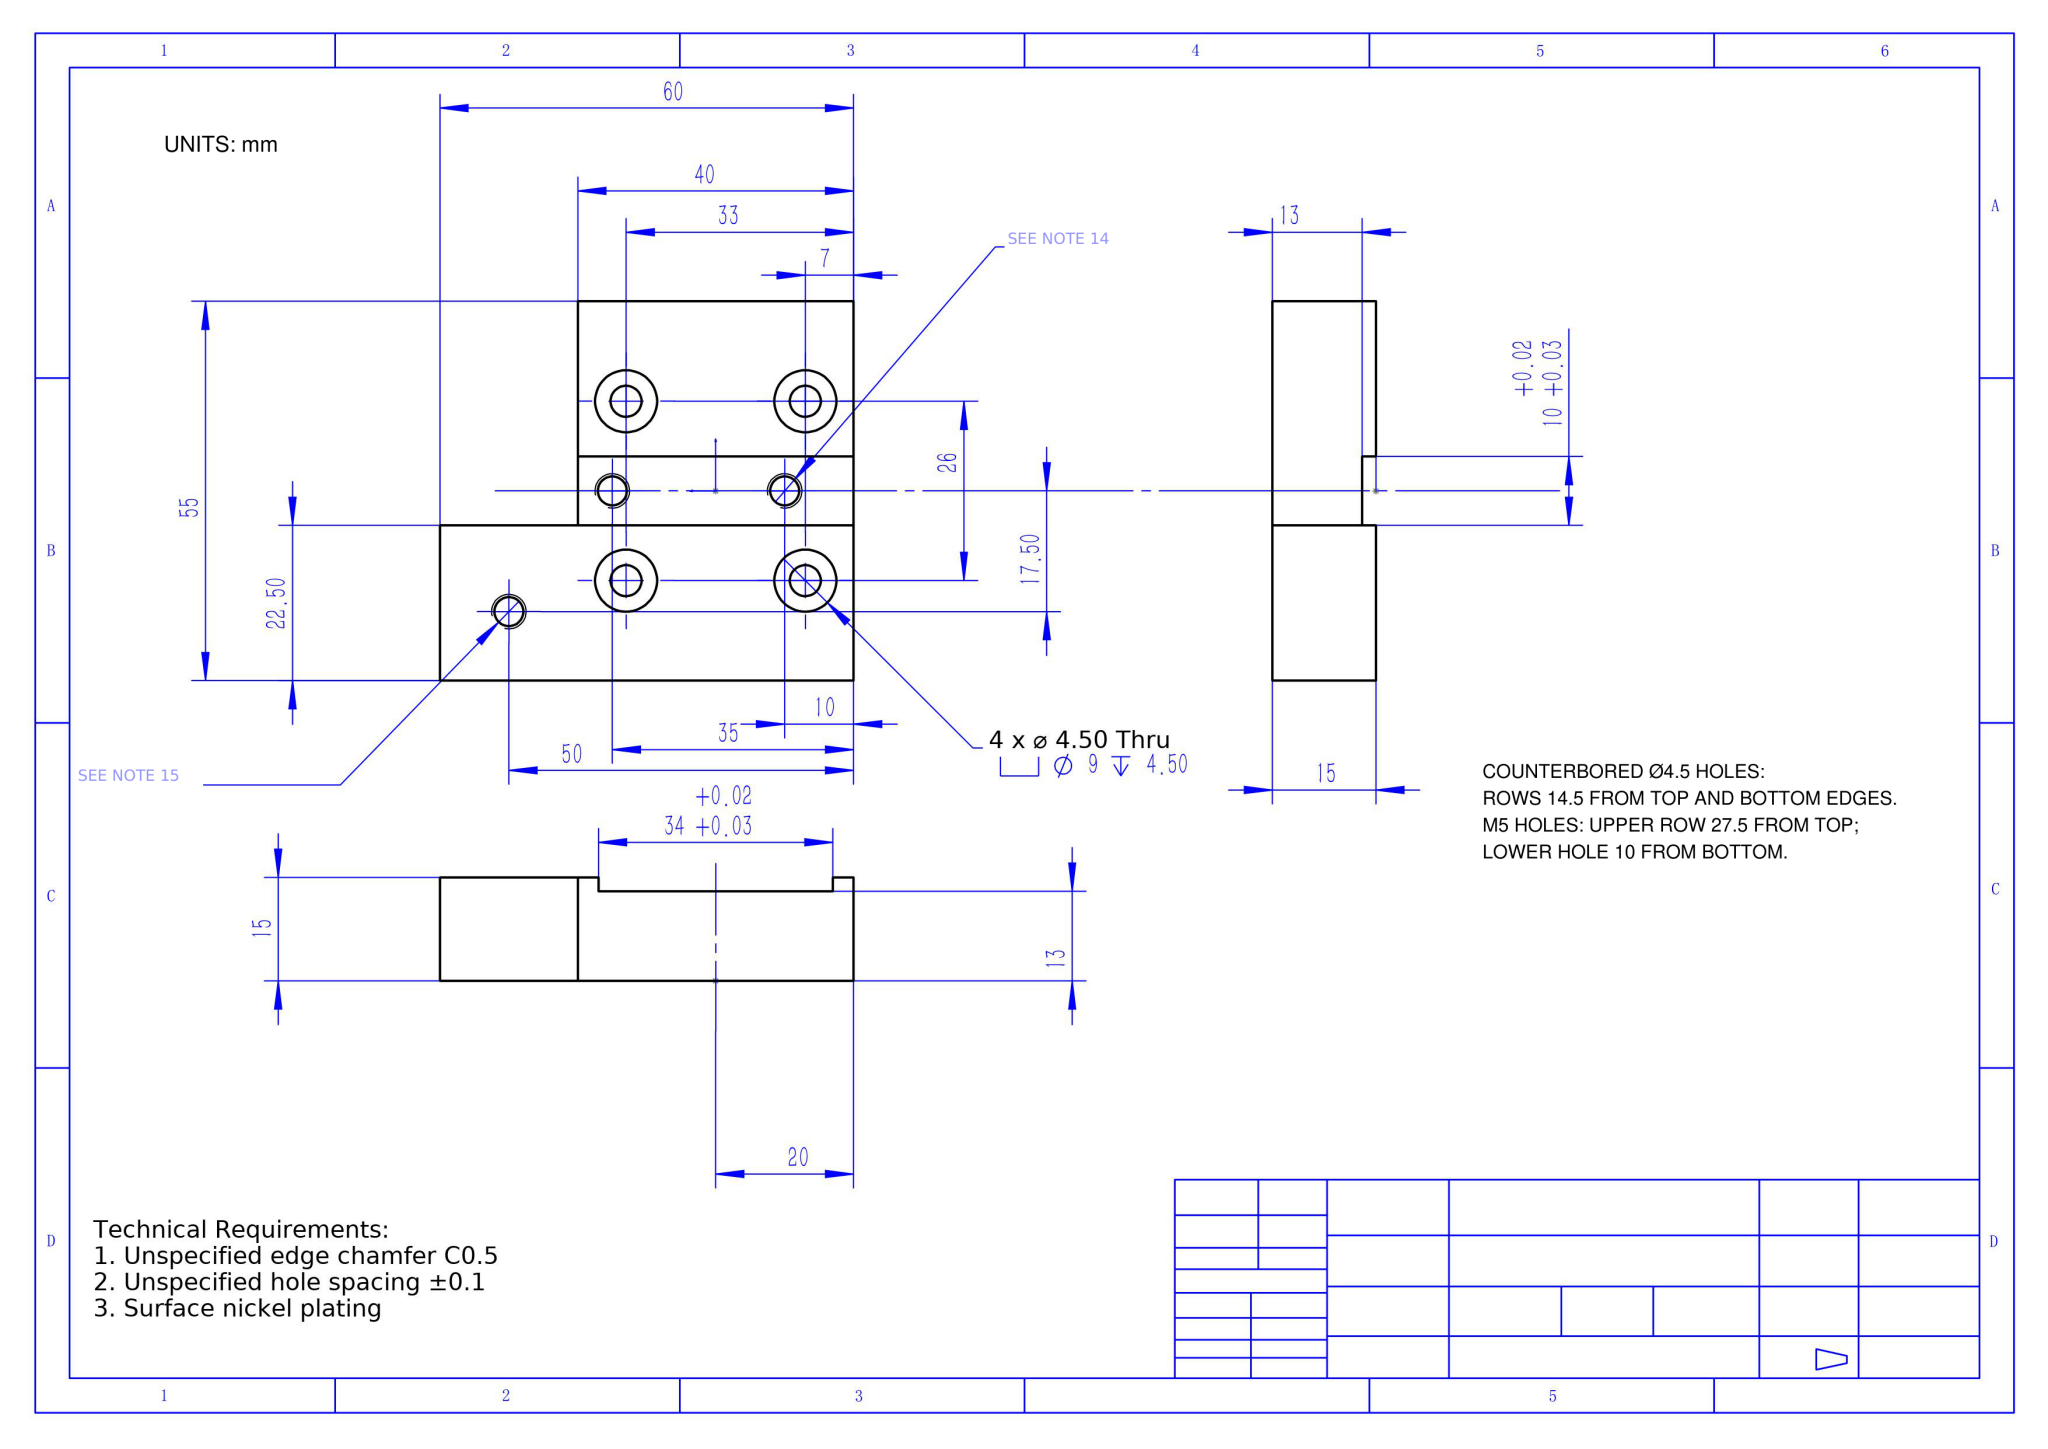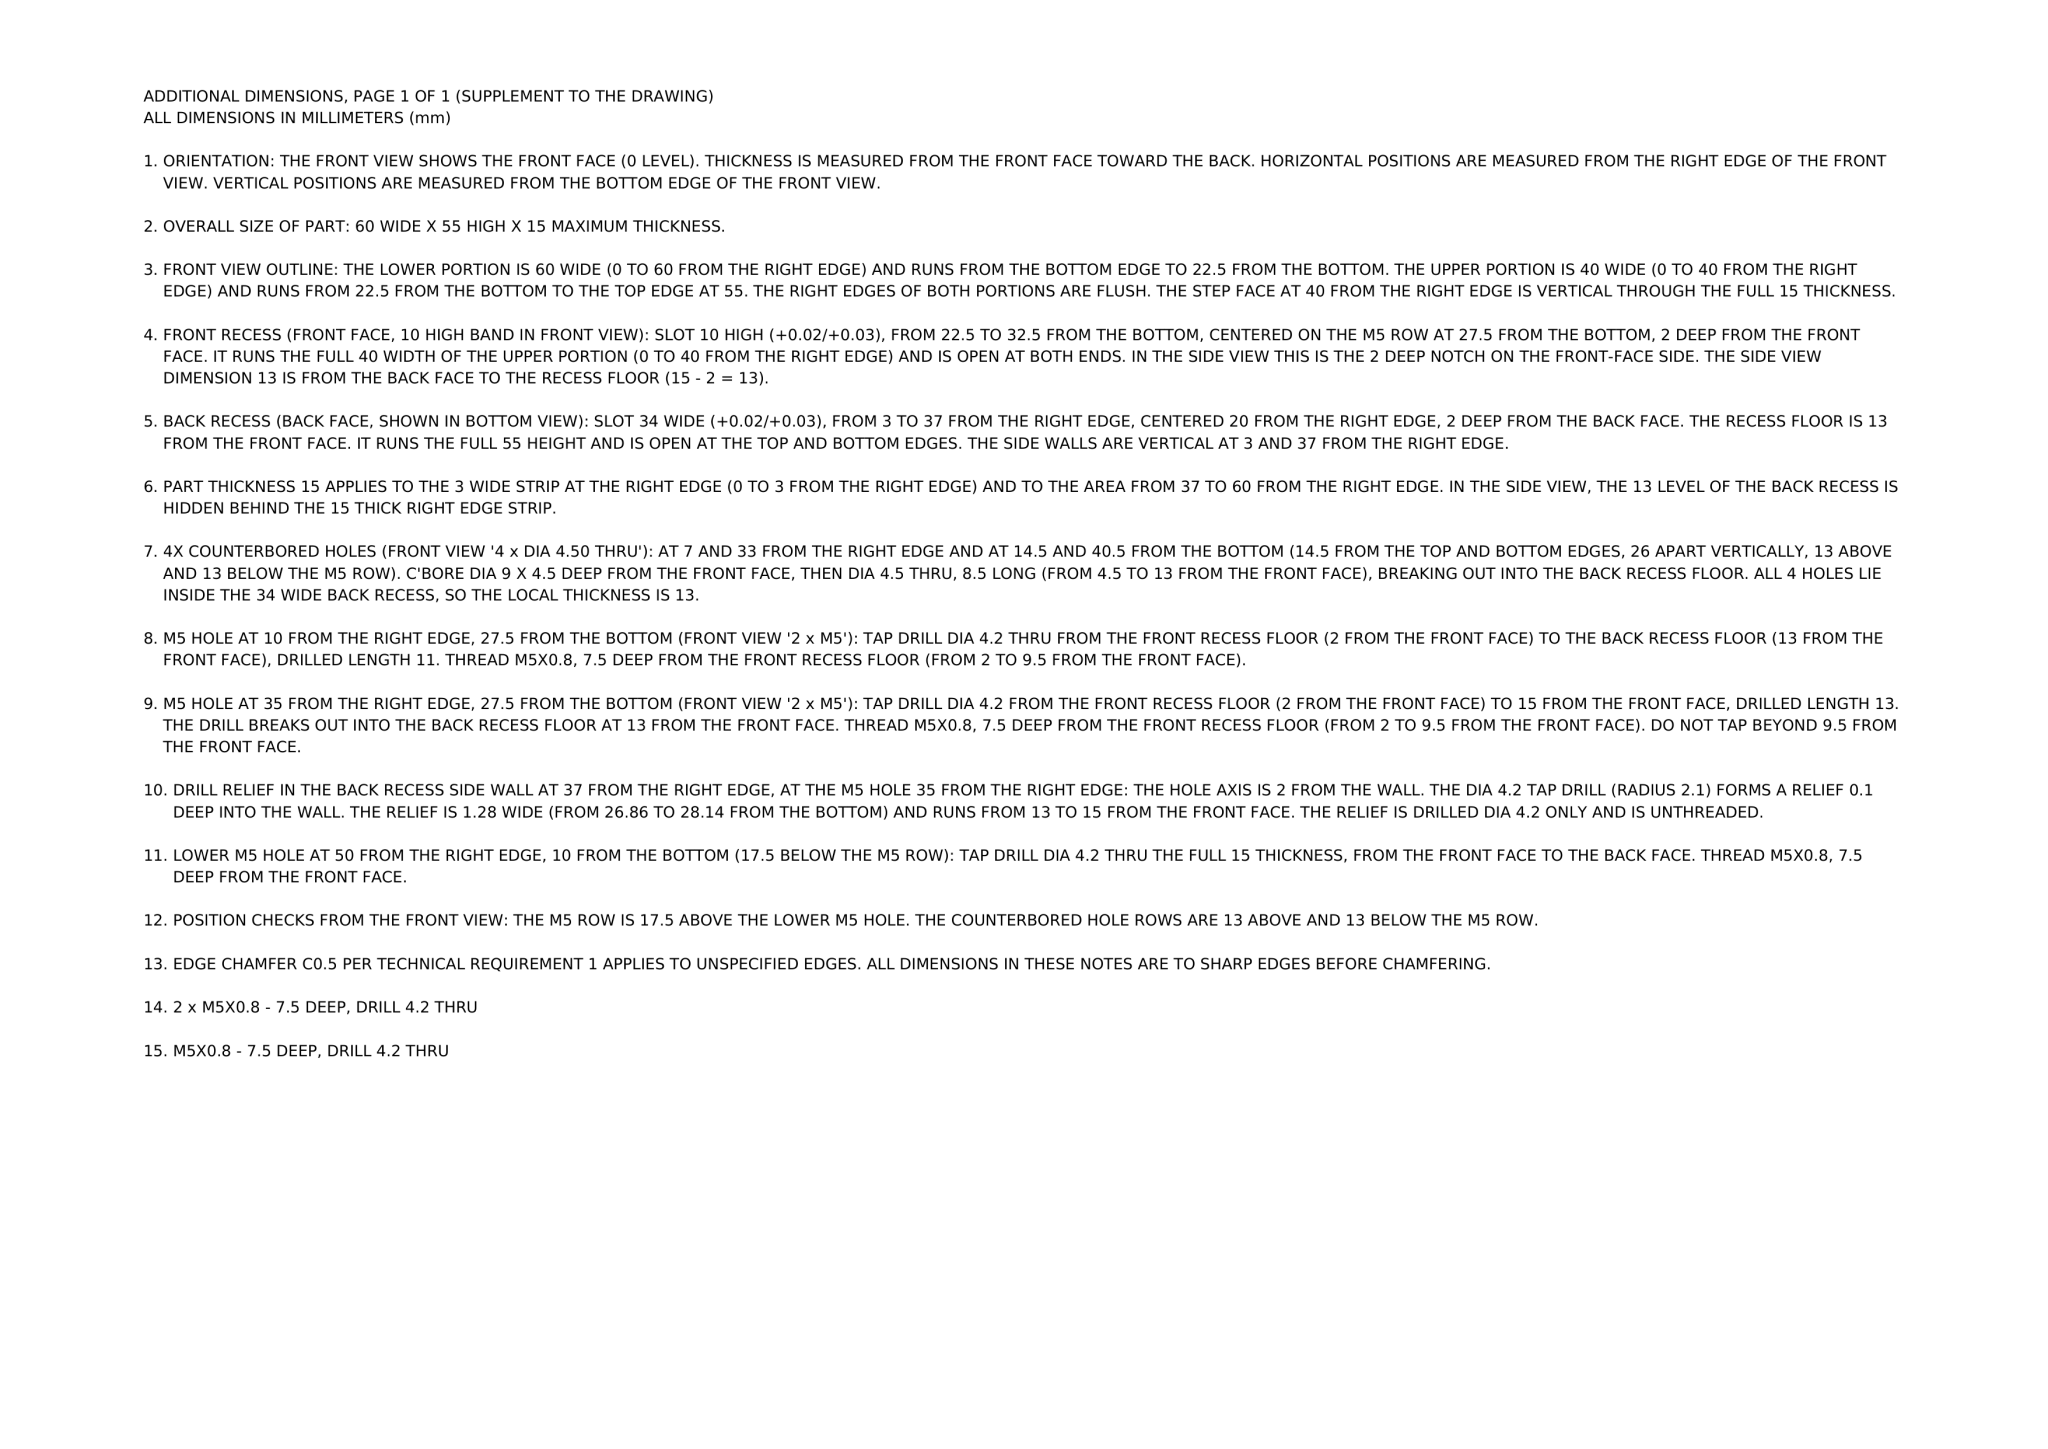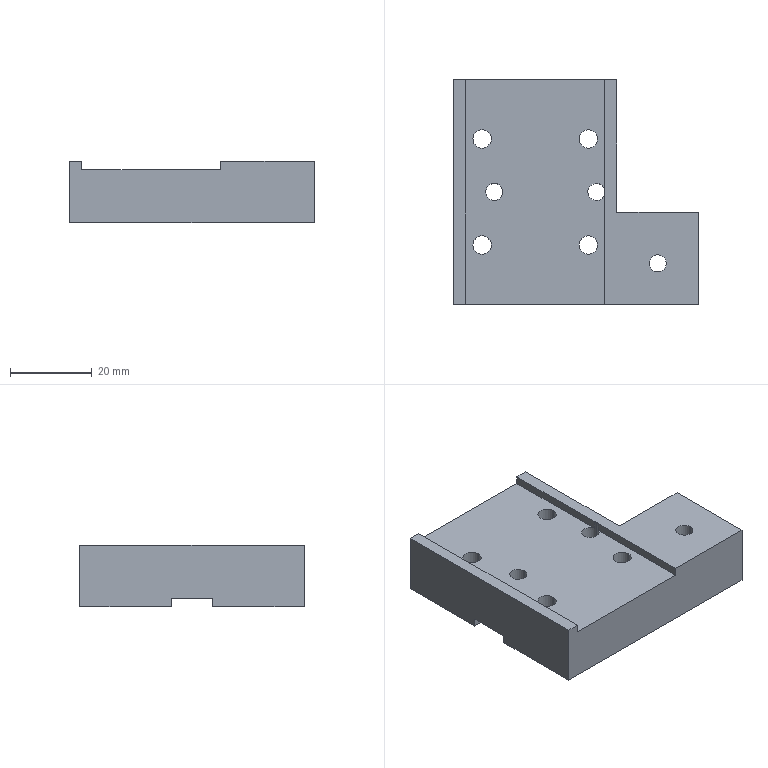Part | NX | mm | 1 solid | 42 faces | box 60 x 55 x 15 mm | volume 33011 mm3 | cylinder 22 | plane 20 | commonest cylinder face diameters 9 x8 4.5 x8 4.2 x6